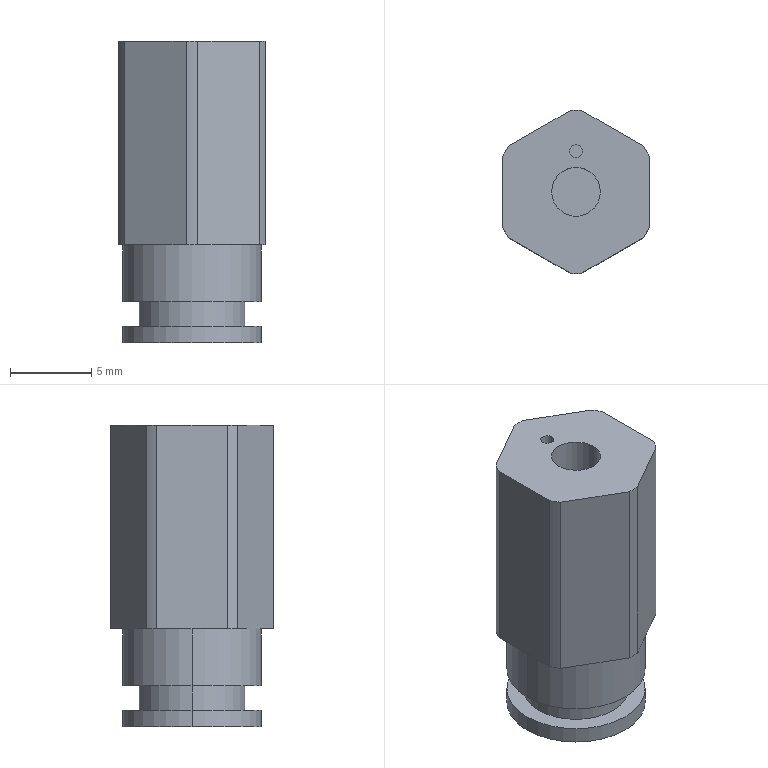Component | SolidWorks | gbgbCJPB6-5-B(0)F8-1_gbgbCJPB6-5_BODYF8-1 | 1 solid | 38 faces | box 9 x 10 x 18.5 mm | volume 878 mm3 | cylinder 20 | plane 14 | cone 4 | commonest cylinder face diameters 10 x6 8.5 x4 0.8 x2 4.134 x2 6 x2 3 x2 6.5 x2
build123d program:
from build123d import *

# Parameters (mm, degrees)
HOLE1_D            = 4.134
HOLE1_DEPTH        = 5
HOLE1_CSINK_D      = 5
HOLE1_CSINK_ANGLE  = 90
HOLE1_TIP          = 1.193
SKETCH5_R          = 23.959
CUT_EXTRUDE1_DEPTH = 12.5
HOLE2_D            = 0.8
HOLE2_DEPTH        = 2


with BuildPart() as part:
    # Sketch1 → Revolve1 (revolve)
    with BuildSketch(Plane.XY, mode=Mode.PRIVATE) as revolve1_sk:
        Polygon((0, 0), (0, 5), (12.5, 5), (12.5, 4.25), (16, 4.25), (16, 3.25), (17.5, 3.25), (17.5, 4.25), (18.5, 4.25), (18.5, 0), align=None)
    revolve(revolve1_sk.sketch.rotate(Axis((18.5, 0, 0), (-1, 0, 0)), 270), axis=Axis((18.5, 0, 0), (-1, 0, 0)))

    # Sketch2 → Cut-Revolve1 (revolve, cut)
    with BuildSketch(Plane.XY, mode=Mode.PRIVATE) as cut_revolve1_sk:
        Polygon((0, 0), (0, 1.5), (3.75, 1.5), (3.75, 3), (10.75, 3), (10.75, 0), align=None)
    revolve(cut_revolve1_sk.sketch.rotate(Axis((10.75, 0, 0), (-1, 0, 0)), 270), axis=Axis((10.75, 0, 0), (-1, 0, 0)), mode=Mode.SUBTRACT)

    # Hole1
    with Locations(Plane(origin=(18.5, 0, 0), x_dir=(0, 0, -1), z_dir=(1, 0, 0))):
        with Locations((0, 0)):
            CounterSinkHole(HOLE1_D / 2, HOLE1_CSINK_D / 2, depth=HOLE1_DEPTH, counter_sink_angle=HOLE1_CSINK_ANGLE)
            with Locations((0, 0, -(HOLE1_DEPTH + HOLE1_TIP / 2))):  # 120° drill point
                Cone(0, HOLE1_D / 2, HOLE1_TIP, mode=Mode.SUBTRACT)

    # Sketch5 → Cut-Extrude1 (cut)
    with BuildSketch(Plane(origin=(0, 0, 0), x_dir=(0, 0, -1), z_dir=(1, 0, 0))):
        Circle(SKETCH5_R)
        Polygon((-4.5, 2.598), (-4.5, -2.598), (0, -5.196), (4.5, -2.598), (4.5, 2.598), (0, 5.196), align=None, mode=Mode.SUBTRACT)
    extrude(amount=CUT_EXTRUDE1_DEPTH, mode=Mode.SUBTRACT)

    # Hole2
    with Locations(Plane.ZY):
        with Locations((0, 2.5)):
            Hole(HOLE2_D / 2, depth=HOLE2_DEPTH)


solid = part.part

# Placed as in the assembly
solid = solid.moved(Location((61.196, 359.97, 412.732), (0, 90, 0)))
STEP:
#1=COLOUR_RGB('',0.7922,0.8196,0.9333);
#2=FILL_AREA_STYLE_COLOUR('',#1);
#3=FILL_AREA_STYLE('',(#2));
#4=SURFACE_STYLE_FILL_AREA(#3);
#5=SURFACE_SIDE_STYLE('',(#4));
#6=SURFACE_STYLE_USAGE(.BOTH.,#5);
#7=PRESENTATION_STYLE_ASSIGNMENT((#6));
#8=CARTESIAN_POINT('',(2.394,14.27,16.171));
#9=VERTEX_POINT('',#8);
#10=CARTESIAN_POINT('',(2.425,14.27,16.171));
#11=VERTEX_POINT('',#10);
#12=CARTESIAN_POINT('',(2.409,14.27,16.171));
#13=DIRECTION('',(0.,0.,1.));
#14=DIRECTION('',(1.,0.,0.));
#15=AXIS2_PLACEMENT_3D('',#12,#13,#14);
#16=CIRCLE('',#15,0.01575);
#17=EDGE_CURVE('',#9,#11,#16,.T.);
#18=ORIENTED_EDGE('',*,*,#17,.F.);
#19=CARTESIAN_POINT('',(2.394,14.27,16.249));
#20=VERTEX_POINT('',#19);
#21=CARTESIAN_POINT('',(2.394,14.27,16.249));
#22=DIRECTION('',(0.,0.,1.));
#23=VECTOR('',#22,39.37);
#24=LINE('',#21,#23);
#25=EDGE_CURVE('',#9,#20,#24,.T.);
#26=ORIENTED_EDGE('',*,*,#25,.T.);
#27=CARTESIAN_POINT('',(2.425,14.27,16.249));
#28=VERTEX_POINT('',#27);
#29=CARTESIAN_POINT('',(2.409,14.27,16.249));
#30=DIRECTION('',(0.,0.,1.));
#31=DIRECTION('',(1.,0.,0.));
#32=AXIS2_PLACEMENT_3D('',#29,#30,#31);
#33=CIRCLE('',#32,0.01575);
#34=EDGE_CURVE('',#20,#28,#33,.T.);
#35=ORIENTED_EDGE('',*,*,#34,.T.);
#36=CARTESIAN_POINT('',(2.425,14.27,16.249));
#37=DIRECTION('',(0.,0.,1.));
#38=VECTOR('',#37,39.37);
#39=LINE('',#36,#38);
#40=EDGE_CURVE('',#11,#28,#39,.T.);
#41=ORIENTED_EDGE('',*,*,#40,.F.);
#42=EDGE_LOOP('',(#18,#26,#35,#41));
#43=FACE_OUTER_BOUND('',#42,.T.);
#44=CARTESIAN_POINT('',(2.409,14.27,16.249));
#45=DIRECTION('',(0.,0.,1.));
#46=DIRECTION('',(1.,0.,0.));
#47=AXIS2_PLACEMENT_3D('',#44,#45,#46);
#48=CYLINDRICAL_SURFACE('',#47,0.01575);
#49=ADVANCED_FACE('',(#43),#48,.F.);
#50=CARTESIAN_POINT('',(2.491,14.172,15.538));
#51=VERTEX_POINT('',#50);
#52=CARTESIAN_POINT('',(2.328,14.172,15.538));
#53=VERTEX_POINT('',#52);
#54=CARTESIAN_POINT('',(2.409,14.172,15.538));
#55=DIRECTION('',(0.,-0.,-1.));
#56=DIRECTION('',(-1.,0.,0.));
#57=AXIS2_PLACEMENT_3D('',#54,#55,#56);
#58=CIRCLE('',#57,0.08138);
#59=EDGE_CURVE('',#51,#53,#58,.T.);
#60=ORIENTED_EDGE('',*,*,#59,.F.);
#61=CARTESIAN_POINT('',(2.508,14.172,15.521));
#62=VERTEX_POINT('',#61);
#63=CARTESIAN_POINT('',(2.508,14.172,15.521));
#64=DIRECTION('',(0.7071,-0.,-0.7071));
#65=VECTOR('',#64,39.37);
#66=LINE('',#63,#65);
#67=EDGE_CURVE('',#51,#62,#66,.T.);
#68=ORIENTED_EDGE('',*,*,#67,.T.);
#69=CARTESIAN_POINT('',(2.311,14.172,15.521));
#70=VERTEX_POINT('',#69);
#71=CARTESIAN_POINT('',(2.409,14.172,15.521));
#72=DIRECTION('',(0.,-0.,-1.));
#73=DIRECTION('',(-1.,0.,0.));
#74=AXIS2_PLACEMENT_3D('',#71,#72,#73);
#75=CIRCLE('',#74,0.09843);
#76=EDGE_CURVE('',#62,#70,#75,.T.);
#77=ORIENTED_EDGE('',*,*,#76,.T.);
#78=CARTESIAN_POINT('',(2.311,14.172,15.521));
#79=DIRECTION('',(-0.7071,-0.,-0.7071));
#80=VECTOR('',#79,39.37);
#81=LINE('',#78,#80);
#82=EDGE_CURVE('',#53,#70,#81,.T.);
#83=ORIENTED_EDGE('',*,*,#82,.F.);
#84=EDGE_LOOP('',(#60,#68,#77,#83));
#85=FACE_OUTER_BOUND('',#84,.T.);
#86=CARTESIAN_POINT('',(2.409,14.172,15.521));
#87=DIRECTION('',(0.,-0.,-1.));
#88=DIRECTION('',(-1.,0.,0.));
#89=AXIS2_PLACEMENT_3D('',#86,#87,#88);
#90=CONICAL_SURFACE('',#89,0.09843,0.7854);
#91=ADVANCED_FACE('',(#85),#90,.F.);
#92=CARTESIAN_POINT('',(2.491,14.172,15.718));
#93=VERTEX_POINT('',#92);
#94=CARTESIAN_POINT('',(2.328,14.172,15.718));
#95=VERTEX_POINT('',#94);
#96=CARTESIAN_POINT('',(2.409,14.172,15.718));
#97=DIRECTION('',(0.,-0.,-1.));
#98=DIRECTION('',(-1.,0.,0.));
#99=AXIS2_PLACEMENT_3D('',#96,#97,#98);
#100=CIRCLE('',#99,0.08138);
#101=EDGE_CURVE('',#93,#95,#100,.T.);
#102=ORIENTED_EDGE('',*,*,#101,.F.);
#103=CARTESIAN_POINT('',(2.491,14.172,15.521));
#104=DIRECTION('',(0.,-0.,-1.));
#105=VECTOR('',#104,39.37);
#106=LINE('',#103,#105);
#107=EDGE_CURVE('',#93,#51,#106,.T.);
#108=ORIENTED_EDGE('',*,*,#107,.T.);
#109=ORIENTED_EDGE('',*,*,#59,.T.);
#110=CARTESIAN_POINT('',(2.328,14.172,15.521));
#111=DIRECTION('',(0.,-0.,-1.));
#112=VECTOR('',#111,39.37);
#113=LINE('',#110,#112);
#114=EDGE_CURVE('',#95,#53,#113,.T.);
#115=ORIENTED_EDGE('',*,*,#114,.F.);
#116=EDGE_LOOP('',(#102,#108,#109,#115));
#117=FACE_OUTER_BOUND('',#116,.T.);
#118=CARTESIAN_POINT('',(2.409,14.172,15.521));
#119=DIRECTION('',(0.,-0.,-1.));
#120=DIRECTION('',(-1.,0.,0.));
#121=AXIS2_PLACEMENT_3D('',#118,#119,#120);
#122=CYLINDRICAL_SURFACE('',#121,0.08138);
#123=ADVANCED_FACE('',(#117),#122,.F.);
#124=CARTESIAN_POINT('',(2.409,14.172,15.765));
#125=VERTEX_POINT('',#124);
#126=CARTESIAN_POINT('',(2.328,14.172,15.718));
#127=DIRECTION('',(-0.866,0.,-0.5));
#128=VECTOR('',#127,39.37);
#129=LINE('',#126,#128);
#130=EDGE_CURVE('',#125,#95,#129,.T.);
#131=ORIENTED_EDGE('',*,*,#130,.F.);
#132=CARTESIAN_POINT('',(2.491,14.172,15.718));
#133=DIRECTION('',(0.866,-0.,-0.5));
#134=VECTOR('',#133,39.37);
#135=LINE('',#132,#134);
#136=EDGE_CURVE('',#125,#93,#135,.T.);
#137=ORIENTED_EDGE('',*,*,#136,.T.);
#138=ORIENTED_EDGE('',*,*,#101,.T.);
#139=EDGE_LOOP('',(#131,#137,#138));
#140=FACE_OUTER_BOUND('',#139,.T.);
#141=CARTESIAN_POINT('',(2.409,14.172,15.718));
#142=DIRECTION('',(0.,-0.,-1.));
#143=DIRECTION('',(-1.,0.,0.));
#144=AXIS2_PLACEMENT_3D('',#141,#142,#143);
#145=CONICAL_SURFACE('',#144,0.08138,1.047);
#146=ADVANCED_FACE('',(#140),#145,.F.);
#147=CARTESIAN_POINT('',(2.291,14.172,15.826));
#148=VERTEX_POINT('',#147);
#149=CARTESIAN_POINT('',(2.527,14.172,15.826));
#150=VERTEX_POINT('',#149);
#151=CARTESIAN_POINT('',(2.409,14.172,15.826));
#152=DIRECTION('',(0.,0.,1.));
#153=DIRECTION('',(1.,0.,0.));
#154=AXIS2_PLACEMENT_3D('',#151,#152,#153);
#155=CIRCLE('',#154,0.1181);
#156=EDGE_CURVE('',#148,#150,#155,.T.);
#157=ORIENTED_EDGE('',*,*,#156,.F.);
#158=CARTESIAN_POINT('',(2.291,14.172,16.102));
#159=VERTEX_POINT('',#158);
#160=CARTESIAN_POINT('',(2.291,14.172,15.826));
#161=DIRECTION('',(0.,0.,1.));
#162=VECTOR('',#161,39.37);
#163=LINE('',#160,#162);
#164=EDGE_CURVE('',#148,#159,#163,.T.);
#165=ORIENTED_EDGE('',*,*,#164,.T.);
#166=CARTESIAN_POINT('',(2.527,14.172,16.102));
#167=VERTEX_POINT('',#166);
#168=CARTESIAN_POINT('',(2.409,14.172,16.102));
#169=DIRECTION('',(0.,0.,1.));
#170=DIRECTION('',(1.,0.,0.));
#171=AXIS2_PLACEMENT_3D('',#168,#169,#170);
#172=CIRCLE('',#171,0.1181);
#173=EDGE_CURVE('',#159,#167,#172,.T.);
#174=ORIENTED_EDGE('',*,*,#173,.T.);
#175=CARTESIAN_POINT('',(2.527,14.172,15.826));
#176=DIRECTION('',(0.,0.,1.));
#177=VECTOR('',#176,39.37);
#178=LINE('',#175,#177);
#179=EDGE_CURVE('',#150,#167,#178,.T.);
#180=ORIENTED_EDGE('',*,*,#179,.F.);
#181=EDGE_LOOP('',(#157,#165,#174,#180));
#182=FACE_OUTER_BOUND('',#181,.T.);
#183=CARTESIAN_POINT('',(2.409,14.172,15.826));
#184=DIRECTION('',(0.,0.,1.));
#185=DIRECTION('',(1.,0.,0.));
#186=AXIS2_PLACEMENT_3D('',#183,#184,#185);
#187=CYLINDRICAL_SURFACE('',#186,0.1181);
#188=ADVANCED_FACE('',(#182),#187,.F.);
#189=CARTESIAN_POINT('',(2.35,14.172,16.102));
#190=VERTEX_POINT('',#189);
#191=CARTESIAN_POINT('',(2.468,14.172,16.102));
#192=VERTEX_POINT('',#191);
#193=CARTESIAN_POINT('',(2.409,14.172,16.102));
#194=DIRECTION('',(0.,0.,1.));
#195=DIRECTION('',(1.,0.,0.));
#196=AXIS2_PLACEMENT_3D('',#193,#194,#195);
#197=CIRCLE('',#196,0.05906);
#198=EDGE_CURVE('',#190,#192,#197,.T.);
#199=ORIENTED_EDGE('',*,*,#198,.F.);
#200=CARTESIAN_POINT('',(2.35,14.172,16.249));
#201=VERTEX_POINT('',#200);
#202=CARTESIAN_POINT('',(2.35,14.172,15.826));
#203=DIRECTION('',(0.,0.,1.));
#204=VECTOR('',#203,39.37);
#205=LINE('',#202,#204);
#206=EDGE_CURVE('',#190,#201,#205,.T.);
#207=ORIENTED_EDGE('',*,*,#206,.T.);
#208=CARTESIAN_POINT('',(2.468,14.172,16.249));
#209=VERTEX_POINT('',#208);
#210=CARTESIAN_POINT('',(2.409,14.172,16.249));
#211=DIRECTION('',(0.,0.,1.));
#212=DIRECTION('',(1.,0.,0.));
#213=AXIS2_PLACEMENT_3D('',#210,#211,#212);
#214=CIRCLE('',#213,0.05906);
#215=EDGE_CURVE('',#201,#209,#214,.T.);
#216=ORIENTED_EDGE('',*,*,#215,.T.);
#217=CARTESIAN_POINT('',(2.468,14.172,15.826));
#218=DIRECTION('',(0.,0.,1.));
#219=VECTOR('',#218,39.37);
#220=LINE('',#217,#219);
#221=EDGE_CURVE('',#192,#209,#220,.T.);
#222=ORIENTED_EDGE('',*,*,#221,.F.);
#223=EDGE_LOOP('',(#199,#207,#216,#222));
#224=FACE_OUTER_BOUND('',#223,.T.);
#225=CARTESIAN_POINT('',(2.409,14.172,15.826));
#226=DIRECTION('',(0.,0.,1.));
#227=DIRECTION('',(1.,0.,0.));
#228=AXIS2_PLACEMENT_3D('',#225,#226,#227);
#229=CYLINDRICAL_SURFACE('',#228,0.05906);
#230=ADVANCED_FACE('',(#224),#229,.F.);
#231=CARTESIAN_POINT('',(2.577,14.172,15.521));
#232=VERTEX_POINT('',#231);
#233=CARTESIAN_POINT('',(2.242,14.172,15.521));
#234=VERTEX_POINT('',#233);
#235=CARTESIAN_POINT('',(2.409,14.172,15.521));
#236=DIRECTION('',(0.,0.,1.));
#237=DIRECTION('',(1.,0.,0.));
#238=AXIS2_PLACEMENT_3D('',#235,#236,#237);
#239=CIRCLE('',#238,0.1673);
#240=EDGE_CURVE('',#232,#234,#239,.T.);
#241=ORIENTED_EDGE('',*,*,#240,.T.);
#242=CARTESIAN_POINT('',(2.242,14.172,15.56));
#243=VERTEX_POINT('',#242);
#244=CARTESIAN_POINT('',(2.242,14.172,15.521));
#245=DIRECTION('',(0.,0.,1.));
#246=VECTOR('',#245,39.37);
#247=LINE('',#244,#246);
#248=EDGE_CURVE('',#234,#243,#247,.T.);
#249=ORIENTED_EDGE('',*,*,#248,.T.);
#250=CARTESIAN_POINT('',(2.577,14.172,15.56));
#251=VERTEX_POINT('',#250);
#252=CARTESIAN_POINT('',(2.409,14.172,15.56));
#253=DIRECTION('',(0.,0.,1.));
#254=DIRECTION('',(1.,0.,0.));
#255=AXIS2_PLACEMENT_3D('',#252,#253,#254);
#256=CIRCLE('',#255,0.1673);
#257=EDGE_CURVE('',#251,#243,#256,.T.);
#258=ORIENTED_EDGE('',*,*,#257,.F.);
#259=CARTESIAN_POINT('',(2.577,14.172,15.521));
#260=DIRECTION('',(0.,0.,1.));
#261=VECTOR('',#260,39.37);
#262=LINE('',#259,#261);
#263=EDGE_CURVE('',#232,#251,#262,.T.);
#264=ORIENTED_EDGE('',*,*,#263,.F.);
#265=EDGE_LOOP('',(#241,#249,#258,#264));
#266=FACE_OUTER_BOUND('',#265,.T.);
#267=CARTESIAN_POINT('',(2.409,14.172,15.521));
#268=DIRECTION('',(0.,0.,1.));
#269=DIRECTION('',(1.,0.,0.));
#270=AXIS2_PLACEMENT_3D('',#267,#268,#269);
#271=CYLINDRICAL_SURFACE('',#270,0.1673);
#272=ADVANCED_FACE('',(#266),#271,.T.);
#273=CARTESIAN_POINT('',(2.537,14.172,15.56));
#274=VERTEX_POINT('',#273);
#275=CARTESIAN_POINT('',(2.281,14.172,15.56));
#276=VERTEX_POINT('',#275);
#277=CARTESIAN_POINT('',(2.409,14.172,15.56));
#278=DIRECTION('',(0.,0.,1.));
#279=DIRECTION('',(1.,0.,0.));
#280=AXIS2_PLACEMENT_3D('',#277,#278,#279);
#281=CIRCLE('',#280,0.128);
#282=EDGE_CURVE('',#274,#276,#281,.T.);
#283=ORIENTED_EDGE('',*,*,#282,.T.);
#284=CARTESIAN_POINT('',(2.281,14.172,15.619));
#285=VERTEX_POINT('',#284);
#286=CARTESIAN_POINT('',(2.281,14.172,15.521));
#287=DIRECTION('',(0.,0.,1.));
#288=VECTOR('',#287,39.37);
#289=LINE('',#286,#288);
#290=EDGE_CURVE('',#276,#285,#289,.T.);
#291=ORIENTED_EDGE('',*,*,#290,.T.);
#292=CARTESIAN_POINT('',(2.537,14.172,15.619));
#293=VERTEX_POINT('',#292);
#294=CARTESIAN_POINT('',(2.409,14.172,15.619));
#295=DIRECTION('',(0.,0.,1.));
#296=DIRECTION('',(1.,0.,0.));
#297=AXIS2_PLACEMENT_3D('',#294,#295,#296);
#298=CIRCLE('',#297,0.128);
#299=EDGE_CURVE('',#293,#285,#298,.T.);
#300=ORIENTED_EDGE('',*,*,#299,.F.);
#301=CARTESIAN_POINT('',(2.537,14.172,15.521));
#302=DIRECTION('',(0.,0.,1.));
#303=VECTOR('',#302,39.37);
#304=LINE('',#301,#303);
#305=EDGE_CURVE('',#274,#293,#304,.T.);
#306=ORIENTED_EDGE('',*,*,#305,.F.);
#307=EDGE_LOOP('',(#283,#291,#300,#306));
#308=FACE_OUTER_BOUND('',#307,.T.);
#309=CARTESIAN_POINT('',(2.409,14.172,15.521));
#310=DIRECTION('',(0.,0.,1.));
#311=DIRECTION('',(1.,0.,0.));
#312=AXIS2_PLACEMENT_3D('',#309,#310,#311);
#313=CYLINDRICAL_SURFACE('',#312,0.128);
#314=ADVANCED_FACE('',(#308),#313,.T.);
#315=CARTESIAN_POINT('',(2.577,14.172,15.619));
#316=VERTEX_POINT('',#315);
#317=CARTESIAN_POINT('',(2.242,14.172,15.619));
#318=VERTEX_POINT('',#317);
#319=CARTESIAN_POINT('',(2.409,14.172,15.619));
#320=DIRECTION('',(0.,0.,1.));
#321=DIRECTION('',(1.,0.,0.));
#322=AXIS2_PLACEMENT_3D('',#319,#320,#321);
#323=CIRCLE('',#322,0.1673);
#324=EDGE_CURVE('',#316,#318,#323,.T.);
#325=ORIENTED_EDGE('',*,*,#324,.T.);
#326=CARTESIAN_POINT('',(2.242,14.172,15.757));
#327=VERTEX_POINT('',#326);
#328=CARTESIAN_POINT('',(2.242,14.172,15.521));
#329=DIRECTION('',(0.,0.,1.));
#330=VECTOR('',#329,39.37);
#331=LINE('',#328,#330);
#332=EDGE_CURVE('',#318,#327,#331,.T.);
#333=ORIENTED_EDGE('',*,*,#332,.T.);
#334=CARTESIAN_POINT('',(2.577,14.172,15.757));
#335=VERTEX_POINT('',#334);
#336=CARTESIAN_POINT('',(2.409,14.172,15.757));
#337=DIRECTION('',(0.,0.,1.));
#338=DIRECTION('',(1.,0.,0.));
#339=AXIS2_PLACEMENT_3D('',#336,#337,#338);
#340=CIRCLE('',#339,0.1673);
#341=EDGE_CURVE('',#335,#327,#340,.T.);
#342=ORIENTED_EDGE('',*,*,#341,.F.);
#343=CARTESIAN_POINT('',(2.577,14.172,15.521));
#344=DIRECTION('',(0.,0.,1.));
#345=VECTOR('',#344,39.37);
#346=LINE('',#343,#345);
#347=EDGE_CURVE('',#316,#335,#346,.T.);
#348=ORIENTED_EDGE('',*,*,#347,.F.);
#349=EDGE_LOOP('',(#325,#333,#342,#348));
#350=FACE_OUTER_BOUND('',#349,.T.);
#351=CARTESIAN_POINT('',(2.409,14.172,15.521));
#352=DIRECTION('',(0.,0.,1.));
#353=DIRECTION('',(1.,0.,0.));
#354=AXIS2_PLACEMENT_3D('',#351,#352,#353);
#355=CYLINDRICAL_SURFACE('',#354,0.1673);
#356=ADVANCED_FACE('',(#350),#355,.T.);
#357=CARTESIAN_POINT('',(2.586,14.258,15.757));
#358=VERTEX_POINT('',#357);
#359=CARTESIAN_POINT('',(2.572,14.283,15.757));
#360=VERTEX_POINT('',#359);
#361=CARTESIAN_POINT('',(2.409,14.172,15.757));
#362=DIRECTION('',(0.,0.,1.));
#363=DIRECTION('',(1.,0.,0.));
#364=AXIS2_PLACEMENT_3D('',#361,#362,#363);
#365=CIRCLE('',#364,0.1969);
#366=EDGE_CURVE('',#358,#360,#365,.T.);
#367=ORIENTED_EDGE('',*,*,#366,.T.);
#368=CARTESIAN_POINT('',(2.572,14.283,16.249));
#369=VERTEX_POINT('',#368);
#370=CARTESIAN_POINT('',(2.572,14.283,15.521));
#371=DIRECTION('',(0.,0.,1.));
#372=VECTOR('',#371,39.37);
#373=LINE('',#370,#372);
#374=EDGE_CURVE('',#360,#369,#373,.T.);
#375=ORIENTED_EDGE('',*,*,#374,.T.);
#376=CARTESIAN_POINT('',(2.586,14.258,16.249));
#377=VERTEX_POINT('',#376);
#378=CARTESIAN_POINT('',(2.409,14.172,16.249));
#379=DIRECTION('',(0.,0.,1.));
#380=DIRECTION('',(1.,0.,0.));
#381=AXIS2_PLACEMENT_3D('',#378,#379,#380);
#382=CIRCLE('',#381,0.1969);
#383=EDGE_CURVE('',#377,#369,#382,.T.);
#384=ORIENTED_EDGE('',*,*,#383,.F.);
#385=CARTESIAN_POINT('',(2.586,14.258,15.521));
#386=DIRECTION('',(0.,-0.,-1.));
#387=VECTOR('',#386,39.37);
#388=LINE('',#385,#387);
#389=EDGE_CURVE('',#377,#358,#388,.T.);
#390=ORIENTED_EDGE('',*,*,#389,.T.);
#391=EDGE_LOOP('',(#367,#375,#384,#390));
#392=FACE_OUTER_BOUND('',#391,.T.);
#393=CARTESIAN_POINT('',(2.409,14.172,15.521));
#394=DIRECTION('',(0.,0.,1.));
#395=DIRECTION('',(1.,0.,0.));
#396=AXIS2_PLACEMENT_3D('',#393,#394,#395);
#397=CYLINDRICAL_SURFACE('',#396,0.1969);
#398=ADVANCED_FACE('',(#392),#397,.T.);
#399=CARTESIAN_POINT('',(2.572,14.062,15.757));
#400=VERTEX_POINT('',#399);
#401=CARTESIAN_POINT('',(2.586,14.086,15.757));
#402=VERTEX_POINT('',#401);
#403=CARTESIAN_POINT('',(2.409,14.172,15.757));
#404=DIRECTION('',(0.,0.,1.));
#405=DIRECTION('',(1.,0.,0.));
#406=AXIS2_PLACEMENT_3D('',#403,#404,#405);
#407=CIRCLE('',#406,0.1969);
#408=EDGE_CURVE('',#400,#402,#407,.T.);
#409=ORIENTED_EDGE('',*,*,#408,.T.);
#410=CARTESIAN_POINT('',(2.586,14.086,16.249));
#411=VERTEX_POINT('',#410);
#412=CARTESIAN_POINT('',(2.586,14.086,15.521));
#413=DIRECTION('',(0.,0.,1.));
#414=VECTOR('',#413,39.37);
#415=LINE('',#412,#414);
#416=EDGE_CURVE('',#402,#411,#415,.T.);
#417=ORIENTED_EDGE('',*,*,#416,.T.);
#418=CARTESIAN_POINT('',(2.572,14.062,16.249));
#419=VERTEX_POINT('',#418);
#420=CARTESIAN_POINT('',(2.409,14.172,16.249));
#421=DIRECTION('',(0.,0.,1.));
#422=DIRECTION('',(1.,0.,0.));
#423=AXIS2_PLACEMENT_3D('',#420,#421,#422);
#424=CIRCLE('',#423,0.1969);
#425=EDGE_CURVE('',#419,#411,#424,.T.);
#426=ORIENTED_EDGE('',*,*,#425,.F.);
#427=CARTESIAN_POINT('',(2.572,14.062,15.521));
#428=DIRECTION('',(0.,-0.,-1.));
#429=VECTOR('',#428,39.37);
#430=LINE('',#427,#429);
#431=EDGE_CURVE('',#419,#400,#430,.T.);
#432=ORIENTED_EDGE('',*,*,#431,.T.);
#433=EDGE_LOOP('',(#409,#417,#426,#432));
#434=FACE_OUTER_BOUND('',#433,.T.);
#435=CARTESIAN_POINT('',(2.409,14.172,15.521));
#436=DIRECTION('',(0.,0.,1.));
#437=DIRECTION('',(1.,0.,0.));
#438=AXIS2_PLACEMENT_3D('',#435,#436,#437);
#439=CYLINDRICAL_SURFACE('',#438,0.1969);
#440=ADVANCED_FACE('',(#434),#439,.T.);
#441=CARTESIAN_POINT('',(2.395,13.976,15.757));
#442=VERTEX_POINT('',#441);
#443=CARTESIAN_POINT('',(2.424,13.976,15.757));
#444=VERTEX_POINT('',#443);
#445=CARTESIAN_POINT('',(2.409,14.172,15.757));
#446=DIRECTION('',(0.,0.,1.));
#447=DIRECTION('',(1.,0.,0.));
#448=AXIS2_PLACEMENT_3D('',#445,#446,#447);
#449=CIRCLE('',#448,0.1969);
#450=EDGE_CURVE('',#442,#444,#449,.T.);
#451=ORIENTED_EDGE('',*,*,#450,.T.);
#452=CARTESIAN_POINT('',(2.424,13.976,16.249));
#453=VERTEX_POINT('',#452);
#454=CARTESIAN_POINT('',(2.424,13.976,15.521));
#455=DIRECTION('',(0.,0.,1.));
#456=VECTOR('',#455,39.37);
#457=LINE('',#454,#456);
#458=EDGE_CURVE('',#444,#453,#457,.T.);
#459=ORIENTED_EDGE('',*,*,#458,.T.);
#460=CARTESIAN_POINT('',(2.395,13.976,16.249));
#461=VERTEX_POINT('',#460);
#462=CARTESIAN_POINT('',(2.409,14.172,16.249));
#463=DIRECTION('',(0.,0.,1.));
#464=DIRECTION('',(1.,0.,0.));
#465=AXIS2_PLACEMENT_3D('',#462,#463,#464);
#466=CIRCLE('',#465,0.1969);
#467=EDGE_CURVE('',#461,#453,#466,.T.);
#468=ORIENTED_EDGE('',*,*,#467,.F.);
#469=CARTESIAN_POINT('',(2.395,13.976,15.521));
#470=DIRECTION('',(0.,-0.,-1.));
#471=VECTOR('',#470,39.37);
#472=LINE('',#469,#471);
#473=EDGE_CURVE('',#461,#442,#472,.T.);
#474=ORIENTED_EDGE('',*,*,#473,.T.);
#475=EDGE_LOOP('',(#451,#459,#468,#474));
#476=FACE_OUTER_BOUND('',#475,.T.);
#477=CARTESIAN_POINT('',(2.409,14.172,15.521));
#478=DIRECTION('',(0.,0.,1.));
#479=DIRECTION('',(1.,0.,0.));
#480=AXIS2_PLACEMENT_3D('',#477,#478,#479);
#481=CYLINDRICAL_SURFACE('',#480,0.1969);
#482=ADVANCED_FACE('',(#476),#481,.T.);
#483=CARTESIAN_POINT('',(2.232,14.086,15.757));
#484=VERTEX_POINT('',#483);
#485=CARTESIAN_POINT('',(2.246,14.062,15.757));
#486=VERTEX_POINT('',#485);
#487=CARTESIAN_POINT('',(2.409,14.172,15.757));
#488=DIRECTION('',(0.,0.,1.));
#489=DIRECTION('',(1.,0.,0.));
#490=AXIS2_PLACEMENT_3D('',#487,#488,#489);
#491=CIRCLE('',#490,0.1969);
#492=EDGE_CURVE('',#484,#486,#491,.T.);
#493=ORIENTED_EDGE('',*,*,#492,.T.);
#494=CARTESIAN_POINT('',(2.246,14.062,16.249));
#495=VERTEX_POINT('',#494);
#496=CARTESIAN_POINT('',(2.246,14.062,15.521));
#497=DIRECTION('',(0.,0.,1.));
#498=VECTOR('',#497,39.37);
#499=LINE('',#496,#498);
#500=EDGE_CURVE('',#486,#495,#499,.T.);
#501=ORIENTED_EDGE('',*,*,#500,.T.);
#502=CARTESIAN_POINT('',(2.232,14.086,16.249));
#503=VERTEX_POINT('',#502);
#504=CARTESIAN_POINT('',(2.409,14.172,16.249));
#505=DIRECTION('',(0.,0.,1.));
#506=DIRECTION('',(1.,0.,0.));
#507=AXIS2_PLACEMENT_3D('',#504,#505,#506);
#508=CIRCLE('',#507,0.1969);
#509=EDGE_CURVE('',#503,#495,#508,.T.);
#510=ORIENTED_EDGE('',*,*,#509,.F.);
#511=CARTESIAN_POINT('',(2.232,14.086,15.521));
#512=DIRECTION('',(0.,-0.,-1.));
#513=VECTOR('',#512,39.37);
#514=LINE('',#511,#513);
#515=EDGE_CURVE('',#503,#484,#514,.T.);
#516=ORIENTED_EDGE('',*,*,#515,.T.);
#517=EDGE_LOOP('',(#493,#501,#510,#516));
#518=FACE_OUTER_BOUND('',#517,.T.);
#519=CARTESIAN_POINT('',(2.409,14.172,15.521));
#520=DIRECTION('',(0.,0.,1.));
#521=DIRECTION('',(1.,0.,0.));
#522=AXIS2_PLACEMENT_3D('',#519,#520,#521);
#523=CYLINDRICAL_SURFACE('',#522,0.1969);
#524=ADVANCED_FACE('',(#518),#523,.T.);
#525=CARTESIAN_POINT('',(2.246,14.283,15.757));
#526=VERTEX_POINT('',#525);
#527=CARTESIAN_POINT('',(2.232,14.258,15.757));
#528=VERTEX_POINT('',#527);
#529=CARTESIAN_POINT('',(2.409,14.172,15.757));
#530=DIRECTION('',(0.,0.,1.));
#531=DIRECTION('',(1.,0.,0.));
#532=AXIS2_PLACEMENT_3D('',#529,#530,#531);
#533=CIRCLE('',#532,0.1969);
#534=EDGE_CURVE('',#526,#528,#533,.T.);
#535=ORIENTED_EDGE('',*,*,#534,.T.);
#536=CARTESIAN_POINT('',(2.232,14.258,16.249));
#537=VERTEX_POINT('',#536);
#538=CARTESIAN_POINT('',(2.232,14.258,15.521));
#539=DIRECTION('',(0.,0.,1.));
#540=VECTOR('',#539,39.37);
#541=LINE('',#538,#540);
#542=EDGE_CURVE('',#528,#537,#541,.T.);
#543=ORIENTED_EDGE('',*,*,#542,.T.);
#544=CARTESIAN_POINT('',(2.246,14.283,16.249));
#545=VERTEX_POINT('',#544);
#546=CARTESIAN_POINT('',(2.409,14.172,16.249));
#547=DIRECTION('',(0.,0.,1.));
#548=DIRECTION('',(1.,0.,0.));
#549=AXIS2_PLACEMENT_3D('',#546,#547,#548);
#550=CIRCLE('',#549,0.1969);
#551=EDGE_CURVE('',#545,#537,#550,.T.);
#552=ORIENTED_EDGE('',*,*,#551,.F.);
#553=CARTESIAN_POINT('',(2.246,14.283,15.521));
#554=DIRECTION('',(0.,-0.,-1.));
#555=VECTOR('',#554,39.37);
#556=LINE('',#553,#555);
#557=EDGE_CURVE('',#545,#526,#556,.T.);
#558=ORIENTED_EDGE('',*,*,#557,.T.);
#559=EDGE_LOOP('',(#535,#543,#552,#558));
#560=FACE_OUTER_BOUND('',#559,.T.);
#561=CARTESIAN_POINT('',(2.409,14.172,15.521));
#562=DIRECTION('',(0.,0.,1.));
#563=DIRECTION('',(1.,0.,0.));
#564=AXIS2_PLACEMENT_3D('',#561,#562,#563);
#565=CYLINDRICAL_SURFACE('',#564,0.1969);
#566=ADVANCED_FACE('',(#560),#565,.T.);
#567=CARTESIAN_POINT('',(2.409,14.27,16.249));
#568=DIRECTION('',(0.,0.,1.));
#569=DIRECTION('',(1.,0.,0.));
#570=AXIS2_PLACEMENT_3D('',#567,#568,#569);
#571=CIRCLE('',#570,0.01575);
#572=EDGE_CURVE('',#28,#20,#571,.T.);
#573=ORIENTED_EDGE('',*,*,#572,.F.);
#574=ORIENTED_EDGE('',*,*,#34,.F.);
#575=EDGE_LOOP('',(#573,#574));
#576=FACE_BOUND('',#575,.T.);
#577=ORIENTED_EDGE('',*,*,#383,.T.);
#578=CARTESIAN_POINT('',(2.424,14.368,16.249));
#579=VERTEX_POINT('',#578);
#580=CARTESIAN_POINT('',(2.409,14.377,16.249));
#581=DIRECTION('',(0.866,-0.5,0.));
#582=VECTOR('',#581,39.37);
#583=LINE('',#580,#582);
#584=EDGE_CURVE('',#579,#369,#583,.T.);
#585=ORIENTED_EDGE('',*,*,#584,.F.);
#586=CARTESIAN_POINT('',(2.395,14.368,16.249));
#587=VERTEX_POINT('',#586);
#588=CARTESIAN_POINT('',(2.409,14.172,16.249));
#589=DIRECTION('',(0.,0.,1.));
#590=DIRECTION('',(1.,0.,0.));
#591=AXIS2_PLACEMENT_3D('',#588,#589,#590);
#592=CIRCLE('',#591,0.1969);
#593=EDGE_CURVE('',#579,#587,#592,.T.);
#594=ORIENTED_EDGE('',*,*,#593,.T.);
#595=CARTESIAN_POINT('',(2.232,14.274,16.249));
#596=DIRECTION('',(0.866,0.5,-0.));
#597=VECTOR('',#596,39.37);
#598=LINE('',#595,#597);
#599=EDGE_CURVE('',#545,#587,#598,.T.);
#600=ORIENTED_EDGE('',*,*,#599,.F.);
#601=ORIENTED_EDGE('',*,*,#551,.T.);
#602=CARTESIAN_POINT('',(2.232,14.07,16.249));
#603=DIRECTION('',(0.,1.,-0.));
#604=VECTOR('',#603,39.37);
#605=LINE('',#602,#604);
#606=EDGE_CURVE('',#503,#537,#605,.T.);
#607=ORIENTED_EDGE('',*,*,#606,.F.);
#608=ORIENTED_EDGE('',*,*,#509,.T.);
#609=CARTESIAN_POINT('',(2.409,13.967,16.249));
#610=DIRECTION('',(-0.866,0.5,-0.));
#611=VECTOR('',#610,39.37);
#612=LINE('',#609,#611);
#613=EDGE_CURVE('',#461,#495,#612,.T.);
#614=ORIENTED_EDGE('',*,*,#613,.F.);
#615=ORIENTED_EDGE('',*,*,#467,.T.);
#616=CARTESIAN_POINT('',(2.586,14.07,16.249));
#617=DIRECTION('',(-0.866,-0.5,0.));
#618=VECTOR('',#617,39.37);
#619=LINE('',#616,#618);
#620=EDGE_CURVE('',#419,#453,#619,.T.);
#621=ORIENTED_EDGE('',*,*,#620,.F.);
#622=ORIENTED_EDGE('',*,*,#425,.T.);
#623=CARTESIAN_POINT('',(2.586,14.274,16.249));
#624=DIRECTION('',(-0.,-1.,0.));
#625=VECTOR('',#624,39.37);
#626=LINE('',#623,#625);
#627=EDGE_CURVE('',#377,#411,#626,.T.);
#628=ORIENTED_EDGE('',*,*,#627,.F.);
#629=EDGE_LOOP('',(#577,#585,#594,#600,#601,#607,#608,#614,#615,#621,#622,#628));
#630=FACE_OUTER_BOUND('',#629,.T.);
#631=CARTESIAN_POINT('',(2.409,14.172,16.249));
#632=DIRECTION('',(0.,0.,1.));
#633=DIRECTION('',(1.,0.,0.));
#634=AXIS2_PLACEMENT_3D('',#631,#632,#633);
#635=CIRCLE('',#634,0.05906);
#636=EDGE_CURVE('',#209,#201,#635,.T.);
#637=ORIENTED_EDGE('',*,*,#636,.F.);
#638=ORIENTED_EDGE('',*,*,#215,.F.);
#639=EDGE_LOOP('',(#637,#638));
#640=FACE_BOUND('',#639,.T.);
#641=CARTESIAN_POINT('',(2.409,14.172,16.249));
#642=DIRECTION('',(0.,-0.,-1.));
#643=DIRECTION('',(-1.,0.,-0.));
#644=AXIS2_PLACEMENT_3D('',#641,#642,#643);
#645=PLANE('',#644);
#646=ADVANCED_FACE('',(#576,#630,#640),#645,.F.);
#647=ORIENTED_EDGE('',*,*,#593,.F.);
#648=CARTESIAN_POINT('',(2.424,14.368,15.757));
#649=VERTEX_POINT('',#648);
#650=CARTESIAN_POINT('',(2.424,14.368,15.521));
#651=DIRECTION('',(0.,-0.,-1.));
#652=VECTOR('',#651,39.37);
#653=LINE('',#650,#652);
#654=EDGE_CURVE('',#579,#649,#653,.T.);
#655=ORIENTED_EDGE('',*,*,#654,.T.);
#656=CARTESIAN_POINT('',(2.395,14.368,15.757));
#657=VERTEX_POINT('',#656);
#658=CARTESIAN_POINT('',(2.409,14.172,15.757));
#659=DIRECTION('',(0.,0.,1.));
#660=DIRECTION('',(1.,0.,0.));
#661=AXIS2_PLACEMENT_3D('',#658,#659,#660);
#662=CIRCLE('',#661,0.1969);
#663=EDGE_CURVE('',#649,#657,#662,.T.);
#664=ORIENTED_EDGE('',*,*,#663,.T.);
#665=CARTESIAN_POINT('',(2.395,14.368,15.521));
#666=DIRECTION('',(0.,0.,1.));
#667=VECTOR('',#666,39.37);
#668=LINE('',#665,#667);
#669=EDGE_CURVE('',#657,#587,#668,.T.);
#670=ORIENTED_EDGE('',*,*,#669,.T.);
#671=EDGE_LOOP('',(#647,#655,#664,#670));
#672=FACE_OUTER_BOUND('',#671,.T.);
#673=CARTESIAN_POINT('',(2.409,14.172,15.521));
#674=DIRECTION('',(0.,0.,1.));
#675=DIRECTION('',(1.,0.,0.));
#676=AXIS2_PLACEMENT_3D('',#673,#674,#675);
#677=CYLINDRICAL_SURFACE('',#676,0.1969);
#678=ADVANCED_FACE('',(#672),#677,.T.);
#679=ORIENTED_EDGE('',*,*,#663,.F.);
#680=CARTESIAN_POINT('',(2.413,14.375,15.757));
#681=DIRECTION('',(0.866,-0.5,0.));
#682=VECTOR('',#681,39.37);
#683=LINE('',#680,#682);
#684=EDGE_CURVE('',#649,#360,#683,.T.);
#685=ORIENTED_EDGE('',*,*,#684,.T.);
#686=ORIENTED_EDGE('',*,*,#366,.F.);
#687=CARTESIAN_POINT('',(2.586,14.369,15.757));
#688=DIRECTION('',(-0.,-1.,0.));
#689=VECTOR('',#688,39.37);
#690=LINE('',#687,#689);
#691=EDGE_CURVE('',#358,#402,#690,.T.);
#692=ORIENTED_EDGE('',*,*,#691,.T.);
#693=ORIENTED_EDGE('',*,*,#408,.F.);
#694=CARTESIAN_POINT('',(2.583,14.068,15.757));
#695=DIRECTION('',(-0.866,-0.5,0.));
#696=VECTOR('',#695,39.37);
#697=LINE('',#694,#696);
#698=EDGE_CURVE('',#400,#444,#697,.T.);
#699=ORIENTED_EDGE('',*,*,#698,.T.);
#700=ORIENTED_EDGE('',*,*,#450,.F.);
#701=CARTESIAN_POINT('',(2.235,14.068,15.757));
#702=DIRECTION('',(-0.866,0.5,-0.));
#703=VECTOR('',#702,39.37);
#704=LINE('',#701,#703);
#705=EDGE_CURVE('',#442,#486,#704,.T.);
#706=ORIENTED_EDGE('',*,*,#705,.T.);
#707=ORIENTED_EDGE('',*,*,#492,.F.);
#708=CARTESIAN_POINT('',(2.232,14.369,15.757));
#709=DIRECTION('',(0.,1.,-0.));
#710=VECTOR('',#709,39.37);
#711=LINE('',#708,#710);
#712=EDGE_CURVE('',#484,#528,#711,.T.);
#713=ORIENTED_EDGE('',*,*,#712,.T.);
#714=ORIENTED_EDGE('',*,*,#534,.F.);
#715=CARTESIAN_POINT('',(2.406,14.375,15.757));
#716=DIRECTION('',(0.866,0.5,-0.));
#717=VECTOR('',#716,39.37);
#718=LINE('',#715,#717);
#719=EDGE_CURVE('',#526,#657,#718,.T.);
#720=ORIENTED_EDGE('',*,*,#719,.T.);
#721=EDGE_LOOP('',(#679,#685,#686,#692,#693,#699,#700,#706,#707,#713,#714,#720));
#722=FACE_OUTER_BOUND('',#721,.T.);
#723=ORIENTED_EDGE('',*,*,#341,.T.);
#724=CARTESIAN_POINT('',(2.409,14.172,15.757));
#725=DIRECTION('',(0.,0.,1.));
#726=DIRECTION('',(1.,0.,0.));
#727=AXIS2_PLACEMENT_3D('',#724,#725,#726);
#728=CIRCLE('',#727,0.1673);
#729=EDGE_CURVE('',#327,#335,#728,.T.);
#730=ORIENTED_EDGE('',*,*,#729,.T.);
#731=EDGE_LOOP('',(#723,#730));
#732=FACE_BOUND('',#731,.T.);
#733=CARTESIAN_POINT('',(2.409,14.369,15.757));
#734=DIRECTION('',(0.,0.,1.));
#735=DIRECTION('',(1.,-0.,0.));
#736=AXIS2_PLACEMENT_3D('',#733,#734,#735);
#737=PLANE('',#736);
#738=ADVANCED_FACE('',(#722,#732),#737,.F.);
#739=ORIENTED_EDGE('',*,*,#332,.F.);
#740=CARTESIAN_POINT('',(2.409,14.172,15.619));
#741=DIRECTION('',(0.,0.,1.));
#742=DIRECTION('',(1.,0.,0.));
#743=AXIS2_PLACEMENT_3D('',#740,#741,#742);
#744=CIRCLE('',#743,0.1673);
#745=EDGE_CURVE('',#318,#316,#744,.T.);
#746=ORIENTED_EDGE('',*,*,#745,.T.);
#747=ORIENTED_EDGE('',*,*,#347,.T.);
#748=ORIENTED_EDGE('',*,*,#729,.F.);
#749=EDGE_LOOP('',(#739,#746,#747,#748));
#750=FACE_OUTER_BOUND('',#749,.T.);
#751=CARTESIAN_POINT('',(2.409,14.172,15.521));
#752=DIRECTION('',(0.,0.,1.));
#753=DIRECTION('',(1.,0.,0.));
#754=AXIS2_PLACEMENT_3D('',#751,#752,#753);
#755=CYLINDRICAL_SURFACE('',#754,0.1673);
#756=ADVANCED_FACE('',(#750),#755,.T.);
#757=ORIENTED_EDGE('',*,*,#324,.F.);
#758=ORIENTED_EDGE('',*,*,#745,.F.);
#759=EDGE_LOOP('',(#757,#758));
#760=FACE_OUTER_BOUND('',#759,.T.);
#761=ORIENTED_EDGE('',*,*,#299,.T.);
#762=CARTESIAN_POINT('',(2.409,14.172,15.619));
#763=DIRECTION('',(0.,0.,1.));
#764=DIRECTION('',(1.,0.,0.));
#765=AXIS2_PLACEMENT_3D('',#762,#763,#764);
#766=CIRCLE('',#765,0.128);
#767=EDGE_CURVE('',#285,#293,#766,.T.);
#768=ORIENTED_EDGE('',*,*,#767,.T.);
#769=EDGE_LOOP('',(#761,#768));
#770=FACE_BOUND('',#769,.T.);
#771=CARTESIAN_POINT('',(2.409,14.339,15.619));
#772=DIRECTION('',(0.,0.,1.));
#773=DIRECTION('',(1.,-0.,0.));
#774=AXIS2_PLACEMENT_3D('',#771,#772,#773);
#775=PLANE('',#774);
#776=ADVANCED_FACE('',(#760,#770),#775,.F.);
#777=ORIENTED_EDGE('',*,*,#290,.F.);
#778=CARTESIAN_POINT('',(2.409,14.172,15.56));
#779=DIRECTION('',(0.,0.,1.));
#780=DIRECTION('',(1.,0.,0.));
#781=AXIS2_PLACEMENT_3D('',#778,#779,#780);
#782=CIRCLE('',#781,0.128);
#783=EDGE_CURVE('',#276,#274,#782,.T.);
#784=ORIENTED_EDGE('',*,*,#783,.T.);
#785=ORIENTED_EDGE('',*,*,#305,.T.);
#786=ORIENTED_EDGE('',*,*,#767,.F.);
#787=EDGE_LOOP('',(#777,#784,#785,#786));
#788=FACE_OUTER_BOUND('',#787,.T.);
#789=CARTESIAN_POINT('',(2.409,14.172,15.521));
#790=DIRECTION('',(0.,0.,1.));
#791=DIRECTION('',(1.,0.,0.));
#792=AXIS2_PLACEMENT_3D('',#789,#790,#791);
#793=CYLINDRICAL_SURFACE('',#792,0.128);
#794=ADVANCED_FACE('',(#788),#793,.T.);
#795=ORIENTED_EDGE('',*,*,#282,.F.);
#796=ORIENTED_EDGE('',*,*,#783,.F.);
#797=EDGE_LOOP('',(#795,#796));
#798=FACE_BOUND('',#797,.T.);
#799=ORIENTED_EDGE('',*,*,#257,.T.);
#800=CARTESIAN_POINT('',(2.409,14.172,15.56));
#801=DIRECTION('',(0.,0.,1.));
#802=DIRECTION('',(1.,0.,0.));
#803=AXIS2_PLACEMENT_3D('',#800,#801,#802);
#804=CIRCLE('',#803,0.1673);
#805=EDGE_CURVE('',#243,#251,#804,.T.);
#806=ORIENTED_EDGE('',*,*,#805,.T.);
#807=EDGE_LOOP('',(#799,#806));
#808=FACE_OUTER_BOUND('',#807,.T.);
#809=CARTESIAN_POINT('',(2.409,14.3,15.56));
#810=DIRECTION('',(0.,-0.,-1.));
#811=DIRECTION('',(-1.,0.,-0.));
#812=AXIS2_PLACEMENT_3D('',#809,#810,#811);
#813=PLANE('',#812);
#814=ADVANCED_FACE('',(#798,#808),#813,.F.);
#815=ORIENTED_EDGE('',*,*,#248,.F.);
#816=CARTESIAN_POINT('',(2.409,14.172,15.521));
#817=DIRECTION('',(0.,0.,1.));
#818=DIRECTION('',(1.,0.,0.));
#819=AXIS2_PLACEMENT_3D('',#816,#817,#818);
#820=CIRCLE('',#819,0.1673);
#821=EDGE_CURVE('',#234,#232,#820,.T.);
#822=ORIENTED_EDGE('',*,*,#821,.T.);
#823=ORIENTED_EDGE('',*,*,#263,.T.);
#824=ORIENTED_EDGE('',*,*,#805,.F.);
#825=EDGE_LOOP('',(#815,#822,#823,#824));
#826=FACE_OUTER_BOUND('',#825,.T.);
#827=CARTESIAN_POINT('',(2.409,14.172,15.521));
#828=DIRECTION('',(0.,0.,1.));
#829=DIRECTION('',(1.,0.,0.));
#830=AXIS2_PLACEMENT_3D('',#827,#828,#829);
#831=CYLINDRICAL_SURFACE('',#830,0.1673);
#832=ADVANCED_FACE('',(#826),#831,.T.);
#833=CARTESIAN_POINT('',(2.409,14.172,15.521));
#834=DIRECTION('',(0.,-0.,-1.));
#835=DIRECTION('',(-1.,0.,0.));
#836=AXIS2_PLACEMENT_3D('',#833,#834,#835);
#837=CIRCLE('',#836,0.09843);
#838=EDGE_CURVE('',#70,#62,#837,.T.);
#839=ORIENTED_EDGE('',*,*,#838,.F.);
#840=ORIENTED_EDGE('',*,*,#76,.F.);
#841=EDGE_LOOP('',(#839,#840));
#842=FACE_BOUND('',#841,.T.);
#843=ORIENTED_EDGE('',*,*,#240,.F.);
#844=ORIENTED_EDGE('',*,*,#821,.F.);
#845=EDGE_LOOP('',(#843,#844));
#846=FACE_OUTER_BOUND('',#845,.T.);
#847=CARTESIAN_POINT('',(2.409,14.339,15.521));
#848=DIRECTION('',(0.,0.,1.));
#849=DIRECTION('',(1.,-0.,0.));
#850=AXIS2_PLACEMENT_3D('',#847,#848,#849);
#851=PLANE('',#850);
#852=ADVANCED_FACE('',(#842,#846),#851,.F.);
#853=ORIENTED_EDGE('',*,*,#206,.F.);
#854=CARTESIAN_POINT('',(2.409,14.172,16.102));
#855=DIRECTION('',(0.,0.,1.));
#856=DIRECTION('',(1.,0.,0.));
#857=AXIS2_PLACEMENT_3D('',#854,#855,#856);
#858=CIRCLE('',#857,0.05906);
#859=EDGE_CURVE('',#192,#190,#858,.T.);
#860=ORIENTED_EDGE('',*,*,#859,.F.);
#861=ORIENTED_EDGE('',*,*,#221,.T.);
#862=ORIENTED_EDGE('',*,*,#636,.T.);
#863=EDGE_LOOP('',(#853,#860,#861,#862));
#864=FACE_OUTER_BOUND('',#863,.T.);
#865=CARTESIAN_POINT('',(2.409,14.172,15.826));
#866=DIRECTION('',(0.,0.,1.));
#867=DIRECTION('',(1.,0.,0.));
#868=AXIS2_PLACEMENT_3D('',#865,#866,#867);
#869=CYLINDRICAL_SURFACE('',#868,0.05906);
#870=ADVANCED_FACE('',(#864),#869,.F.);
#871=ORIENTED_EDGE('',*,*,#859,.T.);
#872=ORIENTED_EDGE('',*,*,#198,.T.);
#873=EDGE_LOOP('',(#871,#872));
#874=FACE_BOUND('',#873,.T.);
#875=CARTESIAN_POINT('',(2.409,14.172,16.102));
#876=DIRECTION('',(0.,0.,1.));
#877=DIRECTION('',(1.,0.,0.));
#878=AXIS2_PLACEMENT_3D('',#875,#876,#877);
#879=CIRCLE('',#878,0.1181);
#880=EDGE_CURVE('',#167,#159,#879,.T.);
#881=ORIENTED_EDGE('',*,*,#880,.F.);
#882=ORIENTED_EDGE('',*,*,#173,.F.);
#883=EDGE_LOOP('',(#881,#882));
#884=FACE_OUTER_BOUND('',#883,.T.);
#885=CARTESIAN_POINT('',(2.409,14.231,16.102));
#886=DIRECTION('',(0.,-0.,-1.));
#887=DIRECTION('',(-1.,0.,-0.));
#888=AXIS2_PLACEMENT_3D('',#885,#886,#887);
#889=PLANE('',#888);
#890=ADVANCED_FACE('',(#874,#884),#889,.T.);
#891=ORIENTED_EDGE('',*,*,#164,.F.);
#892=CARTESIAN_POINT('',(2.409,14.172,15.826));
#893=DIRECTION('',(0.,0.,1.));
#894=DIRECTION('',(1.,0.,0.));
#895=AXIS2_PLACEMENT_3D('',#892,#893,#894);
#896=CIRCLE('',#895,0.1181);
#897=EDGE_CURVE('',#150,#148,#896,.T.);
#898=ORIENTED_EDGE('',*,*,#897,.F.);
#899=ORIENTED_EDGE('',*,*,#179,.T.);
#900=ORIENTED_EDGE('',*,*,#880,.T.);
#901=EDGE_LOOP('',(#891,#898,#899,#900));
#902=FACE_OUTER_BOUND('',#901,.T.);
#903=CARTESIAN_POINT('',(2.409,14.172,15.826));
#904=DIRECTION('',(0.,0.,1.));
#905=DIRECTION('',(1.,0.,0.));
#906=AXIS2_PLACEMENT_3D('',#903,#904,#905);
#907=CYLINDRICAL_SURFACE('',#906,0.1181);
#908=ADVANCED_FACE('',(#902),#907,.F.);
#909=ORIENTED_EDGE('',*,*,#897,.T.);
#910=ORIENTED_EDGE('',*,*,#156,.T.);
#911=EDGE_LOOP('',(#909,#910));
#912=FACE_OUTER_BOUND('',#911,.T.);
#913=CARTESIAN_POINT('',(2.409,14.29,15.826));
#914=DIRECTION('',(0.,0.,1.));
#915=DIRECTION('',(1.,-0.,0.));
#916=AXIS2_PLACEMENT_3D('',#913,#914,#915);
#917=PLANE('',#916);
#918=ADVANCED_FACE('',(#912),#917,.T.);
#919=ORIENTED_EDGE('',*,*,#136,.F.);
#920=ORIENTED_EDGE('',*,*,#130,.T.);
#921=CARTESIAN_POINT('',(2.409,14.172,15.718));
#922=DIRECTION('',(0.,-0.,-1.));
#923=DIRECTION('',(-1.,0.,0.));
#924=AXIS2_PLACEMENT_3D('',#921,#922,#923);
#925=CIRCLE('',#924,0.08138);
#926=EDGE_CURVE('',#95,#93,#925,.T.);
#927=ORIENTED_EDGE('',*,*,#926,.T.);
#928=EDGE_LOOP('',(#919,#920,#927));
#929=FACE_OUTER_BOUND('',#928,.T.);
#930=CARTESIAN_POINT('',(2.409,14.172,15.718));
#931=DIRECTION('',(0.,-0.,-1.));
#932=DIRECTION('',(-1.,0.,0.));
#933=AXIS2_PLACEMENT_3D('',#930,#931,#932);
#934=CONICAL_SURFACE('',#933,0.08138,1.047);
#935=ADVANCED_FACE('',(#929),#934,.F.);
#936=ORIENTED_EDGE('',*,*,#107,.F.);
#937=ORIENTED_EDGE('',*,*,#926,.F.);
#938=ORIENTED_EDGE('',*,*,#114,.T.);
#939=CARTESIAN_POINT('',(2.409,14.172,15.538));
#940=DIRECTION('',(0.,-0.,-1.));
#941=DIRECTION('',(-1.,0.,0.));
#942=AXIS2_PLACEMENT_3D('',#939,#940,#941);
#943=CIRCLE('',#942,0.08138);
#944=EDGE_CURVE('',#53,#51,#943,.T.);
#945=ORIENTED_EDGE('',*,*,#944,.T.);
#946=EDGE_LOOP('',(#936,#937,#938,#945));
#947=FACE_OUTER_BOUND('',#946,.T.);
#948=CARTESIAN_POINT('',(2.409,14.172,15.521));
#949=DIRECTION('',(0.,-0.,-1.));
#950=DIRECTION('',(-1.,0.,0.));
#951=AXIS2_PLACEMENT_3D('',#948,#949,#950);
#952=CYLINDRICAL_SURFACE('',#951,0.08138);
#953=ADVANCED_FACE('',(#947),#952,.F.);
#954=ORIENTED_EDGE('',*,*,#67,.F.);
#955=ORIENTED_EDGE('',*,*,#944,.F.);
#956=ORIENTED_EDGE('',*,*,#82,.T.);
#957=ORIENTED_EDGE('',*,*,#838,.T.);
#958=EDGE_LOOP('',(#954,#955,#956,#957));
#959=FACE_OUTER_BOUND('',#958,.T.);
#960=CARTESIAN_POINT('',(2.409,14.172,15.521));
#961=DIRECTION('',(0.,-0.,-1.));
#962=DIRECTION('',(-1.,0.,0.));
#963=AXIS2_PLACEMENT_3D('',#960,#961,#962);
#964=CONICAL_SURFACE('',#963,0.09843,0.7854);
#965=ADVANCED_FACE('',(#959),#964,.F.);
#966=ORIENTED_EDGE('',*,*,#719,.F.);
#967=ORIENTED_EDGE('',*,*,#557,.F.);
#968=ORIENTED_EDGE('',*,*,#599,.T.);
#969=ORIENTED_EDGE('',*,*,#669,.F.);
#970=EDGE_LOOP('',(#966,#967,#968,#969));
#971=FACE_OUTER_BOUND('',#970,.T.);
#972=CARTESIAN_POINT('',(2.232,14.274,15.757));
#973=DIRECTION('',(0.5,-0.866,0.));
#974=DIRECTION('',(-0.866,-0.5,0.));
#975=AXIS2_PLACEMENT_3D('',#972,#973,#974);
#976=PLANE('',#975);
#977=ADVANCED_FACE('',(#971),#976,.F.);
#978=ORIENTED_EDGE('',*,*,#712,.F.);
#979=ORIENTED_EDGE('',*,*,#515,.F.);
#980=ORIENTED_EDGE('',*,*,#606,.T.);
#981=ORIENTED_EDGE('',*,*,#542,.F.);
#982=EDGE_LOOP('',(#978,#979,#980,#981));
#983=FACE_OUTER_BOUND('',#982,.T.);
#984=CARTESIAN_POINT('',(2.232,14.07,15.757));
#985=DIRECTION('',(1.,-0.,0.));
#986=DIRECTION('',(0.,-0.,-1.));
#987=AXIS2_PLACEMENT_3D('',#984,#985,#986);
#988=PLANE('',#987);
#989=ADVANCED_FACE('',(#983),#988,.F.);
#990=ORIENTED_EDGE('',*,*,#705,.F.);
#991=ORIENTED_EDGE('',*,*,#473,.F.);
#992=ORIENTED_EDGE('',*,*,#613,.T.);
#993=ORIENTED_EDGE('',*,*,#500,.F.);
#994=EDGE_LOOP('',(#990,#991,#992,#993));
#995=FACE_OUTER_BOUND('',#994,.T.);
#996=CARTESIAN_POINT('',(2.409,13.967,15.757));
#997=DIRECTION('',(0.5,0.866,-0.));
#998=DIRECTION('',(0.866,-0.5,0.));
#999=AXIS2_PLACEMENT_3D('',#996,#997,#998);
#1000=PLANE('',#999);
#1001=ADVANCED_FACE('',(#995),#1000,.F.);
#1002=ORIENTED_EDGE('',*,*,#698,.F.);
#1003=ORIENTED_EDGE('',*,*,#431,.F.);
#1004=ORIENTED_EDGE('',*,*,#620,.T.);
#1005=ORIENTED_EDGE('',*,*,#458,.F.);
#1006=EDGE_LOOP('',(#1002,#1003,#1004,#1005));
#1007=FACE_OUTER_BOUND('',#1006,.T.);
#1008=CARTESIAN_POINT('',(2.586,14.07,15.757));
#1009=DIRECTION('',(-0.5,0.866,-0.));
#1010=DIRECTION('',(0.866,0.5,-0.));
#1011=AXIS2_PLACEMENT_3D('',#1008,#1009,#1010);
#1012=PLANE('',#1011);
#1013=ADVANCED_FACE('',(#1007),#1012,.F.);
#1014=ORIENTED_EDGE('',*,*,#691,.F.);
#1015=ORIENTED_EDGE('',*,*,#389,.F.);
#1016=ORIENTED_EDGE('',*,*,#627,.T.);
#1017=ORIENTED_EDGE('',*,*,#416,.F.);
#1018=EDGE_LOOP('',(#1014,#1015,#1016,#1017));
#1019=FACE_OUTER_BOUND('',#1018,.T.);
#1020=CARTESIAN_POINT('',(2.586,14.274,15.757));
#1021=DIRECTION('',(-1.,0.,-0.));
#1022=DIRECTION('',(0.,0.,1.));
#1023=AXIS2_PLACEMENT_3D('',#1020,#1021,#1022);
#1024=PLANE('',#1023);
#1025=ADVANCED_FACE('',(#1019),#1024,.F.);
#1026=ORIENTED_EDGE('',*,*,#684,.F.);
#1027=ORIENTED_EDGE('',*,*,#654,.F.);
#1028=ORIENTED_EDGE('',*,*,#584,.T.);
#1029=ORIENTED_EDGE('',*,*,#374,.F.);
#1030=EDGE_LOOP('',(#1026,#1027,#1028,#1029));
#1031=FACE_OUTER_BOUND('',#1030,.T.);
#1032=CARTESIAN_POINT('',(2.409,14.377,15.757));
#1033=DIRECTION('',(-0.5,-0.866,0.));
#1034=DIRECTION('',(-0.866,0.5,-0.));
#1035=AXIS2_PLACEMENT_3D('',#1032,#1033,#1034);
#1036=PLANE('',#1035);
#1037=ADVANCED_FACE('',(#1031),#1036,.F.);
#1038=CARTESIAN_POINT('',(2.409,14.27,16.171));
#1039=DIRECTION('',(0.,0.,1.));
#1040=DIRECTION('',(1.,0.,0.));
#1041=AXIS2_PLACEMENT_3D('',#1038,#1039,#1040);
#1042=CIRCLE('',#1041,0.01575);
#1043=EDGE_CURVE('',#11,#9,#1042,.T.);
#1044=ORIENTED_EDGE('',*,*,#1043,.T.);
#1045=ORIENTED_EDGE('',*,*,#17,.T.);
#1046=EDGE_LOOP('',(#1044,#1045));
#1047=FACE_OUTER_BOUND('',#1046,.T.);
#1048=CARTESIAN_POINT('',(2.409,14.27,16.171));
#1049=DIRECTION('',(0.,-0.,-1.));
#1050=DIRECTION('',(-1.,0.,-0.));
#1051=AXIS2_PLACEMENT_3D('',#1048,#1049,#1050);
#1052=PLANE('',#1051);
#1053=ADVANCED_FACE('',(#1047),#1052,.F.);
#1054=ORIENTED_EDGE('',*,*,#25,.F.);
#1055=ORIENTED_EDGE('',*,*,#1043,.F.);
#1056=ORIENTED_EDGE('',*,*,#40,.T.);
#1057=ORIENTED_EDGE('',*,*,#572,.T.);
#1058=EDGE_LOOP('',(#1054,#1055,#1056,#1057));
#1059=FACE_OUTER_BOUND('',#1058,.T.);
#1060=CARTESIAN_POINT('',(2.409,14.27,16.249));
#1061=DIRECTION('',(0.,0.,1.));
#1062=DIRECTION('',(1.,0.,0.));
#1063=AXIS2_PLACEMENT_3D('',#1060,#1061,#1062);
#1064=CYLINDRICAL_SURFACE('',#1063,0.01575);
#1065=ADVANCED_FACE('',(#1059),#1064,.F.);
#1066=CLOSED_SHELL('',(#49,#91,#123,#146,#188,#230,#272,#314,#356,#398,#440,#482,#524,#566,#646,#678,#738,#756,#776,#794,#814,#832,#852,#870,#890,#908,#918,#935,#953,#965,#977,#989,#1001,#1013,#1025,#1037,#1053,#1065));
#1067=MANIFOLD_SOLID_BREP('',#1066);
#1068=STYLED_ITEM('',(#7),#1067);
#1069=PRESENTATION_LAYER_ASSIGNMENT('','',(#1068));
#1070=(LENGTH_UNIT()NAMED_UNIT(*)SI_UNIT($,.METRE.));
#1071=LENGTH_MEASURE_WITH_UNIT(LENGTH_MEASURE(0.0254),#1070);
#1072=DIMENSIONAL_EXPONENTS(1.,0.,0.,0.,0.,0.,0.);
#1073=(CONVERSION_BASED_UNIT('',#1071)LENGTH_UNIT()NAMED_UNIT(#1072));
#1074=UNCERTAINTY_MEASURE_WITH_UNIT(LENGTH_MEASURE(0.00001),#1073,'','');
#1075=(NAMED_UNIT(*)PLANE_ANGLE_UNIT()SI_UNIT($,.RADIAN.));
#1076=(NAMED_UNIT(*)SI_UNIT($,.STERADIAN.)SOLID_ANGLE_UNIT());
#1077=(GEOMETRIC_REPRESENTATION_CONTEXT(3)GLOBAL_UNCERTAINTY_ASSIGNED_CONTEXT((#1074))GLOBAL_UNIT_ASSIGNED_CONTEXT((#1073,#1075,#1076))REPRESENTATION_CONTEXT('',''));
#1078=MECHANICAL_DESIGN_GEOMETRIC_PRESENTATION_REPRESENTATION('',(#1068),#1077);
#1079=CARTESIAN_POINT('',(0.,0.,0.));
#1080=DIRECTION('',(0.,0.,1.));
#1081=DIRECTION('',(1.,0.,0.));
#1082=AXIS2_PLACEMENT_3D('',#1079,#1080,#1081);
#1083=(LENGTH_UNIT()NAMED_UNIT(*)SI_UNIT($,.METRE.));
#1084=LENGTH_MEASURE_WITH_UNIT(LENGTH_MEASURE(0.0254),#1083);
#1085=DIMENSIONAL_EXPONENTS(1.,0.,0.,0.,0.,0.,0.);
#1086=(CONVERSION_BASED_UNIT('',#1084)LENGTH_UNIT()NAMED_UNIT(#1085));
#1087=UNCERTAINTY_MEASURE_WITH_UNIT(LENGTH_MEASURE(0.00001),#1086,'','');
#1088=(NAMED_UNIT(*)PLANE_ANGLE_UNIT()SI_UNIT($,.RADIAN.));
#1089=(NAMED_UNIT(*)SI_UNIT($,.STERADIAN.)SOLID_ANGLE_UNIT());
#1090=(GEOMETRIC_REPRESENTATION_CONTEXT(3)GLOBAL_UNCERTAINTY_ASSIGNED_CONTEXT((#1087))GLOBAL_UNIT_ASSIGNED_CONTEXT((#1086,#1088,#1089))REPRESENTATION_CONTEXT('',''));
#1091=ADVANCED_BREP_SHAPE_REPRESENTATION('',(#1067,#1082),#1090);